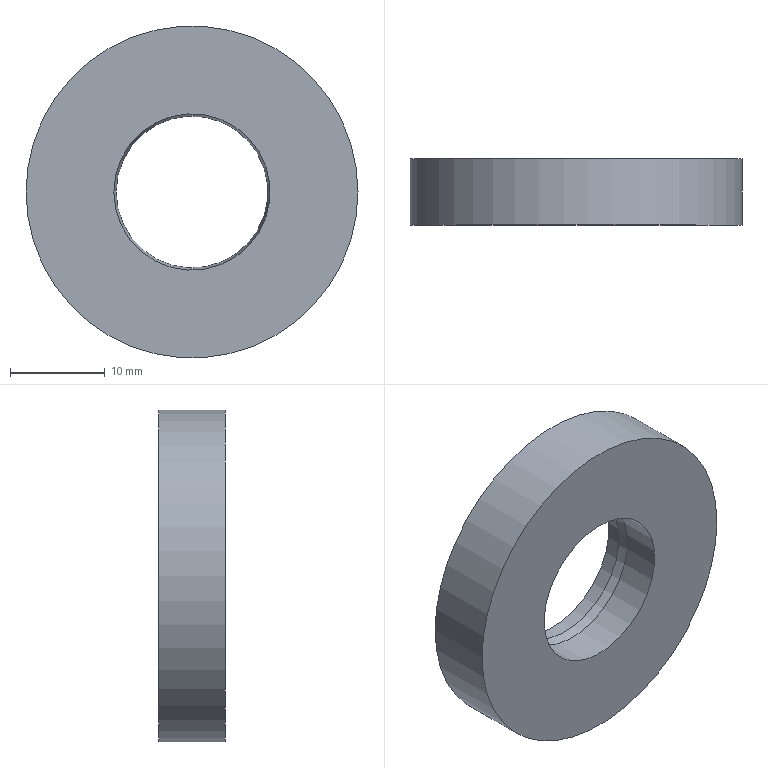Component | NX | OIL_SEAL | 1 solid | 13 faces | box 35 x 7 x 35 mm | volume 2764 mm3 | cylinder 6 | plane 4 | cone 2 | torus 1 | commonest cylinder face diameters 19.32 x2 16.492 x1 35 x1 31.25 x1 16.792 x1
STEP:
#1=CARTESIAN_POINT('',(0.,0.,0.));
#2=DIRECTION('',(0.,0.,1.));
#3=DIRECTION('',(1.,0.,0.));
#4=AXIS2_PLACEMENT_3D('',#1,#2,#3);
#5=CARTESIAN_POINT('',(-8.246,56.,0.));
#6=VERTEX_POINT('',#5);
#7=CARTESIAN_POINT('',(0.,56.,0.));
#8=DIRECTION('',(0.,-1.,0.));
#9=DIRECTION('',(-1.,0.,0.));
#10=AXIS2_PLACEMENT_3D('',#7,#8,#9);
#11=CIRCLE('',#10,8.246);
#12=CARTESIAN_POINT('',(0.,56.,0.));
#13=DIRECTION('',(0.,-1.,0.));
#14=DIRECTION('',(1.,0.,0.));
#15=AXIS2_PLACEMENT_3D('',#12,#13,#14);
#16=CYLINDRICAL_SURFACE('',#15,8.246);
#17=CARTESIAN_POINT('',(3.142,0.));
#18=DIRECTION('',(1.,0.));
#19=VECTOR('',#18,1.);
#20=LINE('',#17,#19);
#21=(GEOMETRIC_REPRESENTATION_CONTEXT(2)PARAMETRIC_REPRESENTATION_CONTEXT()REPRESENTATION_CONTEXT('',''));
#22=DEFINITIONAL_REPRESENTATION('',(#20),#21);
#23=PCURVE('',#16,#22);
#24=CARTESIAN_POINT('',(-8.246,56.,0.));
#25=DIRECTION('',(0.,-1.,0.));
#26=DIRECTION('',(1.,0.,0.));
#27=AXIS2_PLACEMENT_3D('',#24,#25,#26);
#28=PLANE('',#27);
#29=CARTESIAN_POINT('',(8.246,0.));
#30=DIRECTION('',(-1.,0.));
#31=AXIS2_PLACEMENT_2D('',#29,#30);
#32=CIRCLE('',#31,8.246);
#33=(GEOMETRIC_REPRESENTATION_CONTEXT(2)PARAMETRIC_REPRESENTATION_CONTEXT()REPRESENTATION_CONTEXT('',''));
#34=DEFINITIONAL_REPRESENTATION('',(#32),#33);
#35=PCURVE('',#28,#34);
#36=SURFACE_CURVE('',#11,(#23,#35),.PCURVE_S1.);
#37=EDGE_CURVE('',#6,#6,#36,.T.);
#38=ORIENTED_EDGE('',*,*,#37,.F.);
#39=CARTESIAN_POINT('',(-8.246,60.06,0.));
#40=VERTEX_POINT('',#39);
#41=CARTESIAN_POINT('',(-8.246,60.06,0.));
#42=CARTESIAN_POINT('',(-8.246,56.,0.));
#43=B_SPLINE_CURVE_WITH_KNOTS('',1,(#41,#42),.UNSPECIFIED.,.F.,.F.,(2,2),(-4.06,0.),.PIECEWISE_BEZIER_KNOTS.);
#44=CARTESIAN_POINT('',(3.142,0.));
#45=DIRECTION('',(0.,1.));
#46=VECTOR('',#45,1.);
#47=LINE('',#44,#46);
#48=(GEOMETRIC_REPRESENTATION_CONTEXT(2)PARAMETRIC_REPRESENTATION_CONTEXT()REPRESENTATION_CONTEXT('',''));
#49=DEFINITIONAL_REPRESENTATION('',(#47),#48);
#50=PCURVE('',#16,#49);
#51=CARTESIAN_POINT('',(9.425,0.));
#52=DIRECTION('',(0.,1.));
#53=VECTOR('',#52,1.);
#54=LINE('',#51,#53);
#55=(GEOMETRIC_REPRESENTATION_CONTEXT(2)PARAMETRIC_REPRESENTATION_CONTEXT()REPRESENTATION_CONTEXT('',''));
#56=DEFINITIONAL_REPRESENTATION('',(#54),#55);
#57=PCURVE('',#16,#56);
#58=SEAM_CURVE('',#43,(#50,#57),.PCURVE_S1.);
#59=EDGE_CURVE('',#40,#6,#58,.T.);
#60=ORIENTED_EDGE('',*,*,#59,.F.);
#61=CARTESIAN_POINT('',(0.,60.06,0.));
#62=DIRECTION('',(0.,-1.,0.));
#63=DIRECTION('',(-1.,0.,0.));
#64=AXIS2_PLACEMENT_3D('',#61,#62,#63);
#65=CIRCLE('',#64,8.246);
#66=CARTESIAN_POINT('',(3.142,-4.06));
#67=DIRECTION('',(1.,0.));
#68=VECTOR('',#67,1.);
#69=LINE('',#66,#68);
#70=(GEOMETRIC_REPRESENTATION_CONTEXT(2)PARAMETRIC_REPRESENTATION_CONTEXT()REPRESENTATION_CONTEXT('',''));
#71=DEFINITIONAL_REPRESENTATION('',(#69),#70);
#72=PCURVE('',#16,#71);
#73=CARTESIAN_POINT('',(0.,61.106,0.));
#74=DIRECTION('',(0.,-1.,0.));
#75=DIRECTION('',(1.,0.,0.));
#76=AXIS2_PLACEMENT_3D('',#73,#74,#75);
#77=CONICAL_SURFACE('',#76,8.,0.231);
#78=CARTESIAN_POINT('',(3.142,1.046));
#79=DIRECTION('',(1.,0.));
#80=VECTOR('',#79,1.);
#81=LINE('',#78,#80);
#82=(GEOMETRIC_REPRESENTATION_CONTEXT(2)PARAMETRIC_REPRESENTATION_CONTEXT()REPRESENTATION_CONTEXT('',''));
#83=DEFINITIONAL_REPRESENTATION('',(#81),#82);
#84=PCURVE('',#77,#83);
#85=SURFACE_CURVE('',#65,(#72,#84),.PCURVE_S1.);
#86=EDGE_CURVE('',#40,#40,#85,.T.);
#87=ORIENTED_EDGE('',*,*,#86,.T.);
#88=ORIENTED_EDGE('',*,*,#59,.T.);
#89=EDGE_LOOP('',(#38,#60,#87,#88));
#90=FACE_BOUND('',#89,.F.);
#91=ADVANCED_FACE('',(#90),#16,.F.);
#92=CARTESIAN_POINT('',(-17.5,56.,0.));
#93=VERTEX_POINT('',#92);
#94=CARTESIAN_POINT('',(0.,56.,0.));
#95=DIRECTION('',(0.,-1.,0.));
#96=DIRECTION('',(-1.,0.,0.));
#97=AXIS2_PLACEMENT_3D('',#94,#95,#96);
#98=CIRCLE('',#97,17.5);
#99=CARTESIAN_POINT('',(8.246,0.));
#100=DIRECTION('',(-1.,0.));
#101=AXIS2_PLACEMENT_2D('',#99,#100);
#102=CIRCLE('',#101,17.5);
#103=(GEOMETRIC_REPRESENTATION_CONTEXT(2)PARAMETRIC_REPRESENTATION_CONTEXT()REPRESENTATION_CONTEXT('',''));
#104=DEFINITIONAL_REPRESENTATION('',(#102),#103);
#105=PCURVE('',#28,#104);
#106=CARTESIAN_POINT('',(0.,56.,0.));
#107=DIRECTION('',(0.,-1.,0.));
#108=DIRECTION('',(1.,0.,0.));
#109=AXIS2_PLACEMENT_3D('',#106,#107,#108);
#110=CYLINDRICAL_SURFACE('',#109,17.5);
#111=CARTESIAN_POINT('',(3.142,0.));
#112=DIRECTION('',(1.,0.));
#113=VECTOR('',#112,1.);
#114=LINE('',#111,#113);
#115=(GEOMETRIC_REPRESENTATION_CONTEXT(2)PARAMETRIC_REPRESENTATION_CONTEXT()REPRESENTATION_CONTEXT('',''));
#116=DEFINITIONAL_REPRESENTATION('',(#114),#115);
#117=PCURVE('',#110,#116);
#118=SURFACE_CURVE('',#98,(#105,#117),.PCURVE_S1.);
#119=EDGE_CURVE('',#93,#93,#118,.T.);
#120=ORIENTED_EDGE('',*,*,#119,.T.);
#121=EDGE_LOOP('',(#120));
#122=FACE_BOUND('',#121,.T.);
#123=ORIENTED_EDGE('',*,*,#37,.F.);
#124=EDGE_LOOP('',(#123));
#125=FACE_BOUND('',#124,.T.);
#126=ADVANCED_FACE('',(#122,#125),#28,.T.);
#127=CARTESIAN_POINT('',(-17.5,63.,0.));
#128=VERTEX_POINT('',#127);
#129=CARTESIAN_POINT('',(0.,63.,0.));
#130=DIRECTION('',(0.,-1.,0.));
#131=DIRECTION('',(-1.,0.,0.));
#132=AXIS2_PLACEMENT_3D('',#129,#130,#131);
#133=CIRCLE('',#132,17.5);
#134=CARTESIAN_POINT('',(3.142,-7.));
#135=DIRECTION('',(1.,0.));
#136=VECTOR('',#135,1.);
#137=LINE('',#134,#136);
#138=(GEOMETRIC_REPRESENTATION_CONTEXT(2)PARAMETRIC_REPRESENTATION_CONTEXT()REPRESENTATION_CONTEXT('',''));
#139=DEFINITIONAL_REPRESENTATION('',(#137),#138);
#140=PCURVE('',#110,#139);
#141=CARTESIAN_POINT('',(-17.5,63.,0.));
#142=DIRECTION('',(0.,1.,0.));
#143=DIRECTION('',(-1.,0.,0.));
#144=AXIS2_PLACEMENT_3D('',#141,#142,#143);
#145=PLANE('',#144);
#146=CARTESIAN_POINT('',(0.,0.));
#147=CARTESIAN_POINT('',(0.,-30.311));
#148=CARTESIAN_POINT('',(-26.25,-15.155));
#149=CARTESIAN_POINT('',(-52.5,-0.));
#150=CARTESIAN_POINT('',(-26.25,15.155));
#151=CARTESIAN_POINT('',(-0.,30.311));
#152=CARTESIAN_POINT('',(0.,0.));
#153=(BOUNDED_CURVE()B_SPLINE_CURVE(2,(#146,#147,#148,#149,#150,#151,#152),.UNSPECIFIED.,.T.,.F.)B_SPLINE_CURVE_WITH_KNOTS((1,2,2,2,2,1),(-2.094,0.,2.094,4.189,6.283,8.378),.UNSPECIFIED.)CURVE()GEOMETRIC_REPRESENTATION_ITEM()RATIONAL_B_SPLINE_CURVE((1.,0.5,1.,0.5,1.,0.5,1.))REPRESENTATION_ITEM(''));
#154=(GEOMETRIC_REPRESENTATION_CONTEXT(2)PARAMETRIC_REPRESENTATION_CONTEXT()REPRESENTATION_CONTEXT('',''));
#155=DEFINITIONAL_REPRESENTATION('',(#153),#154);
#156=PCURVE('',#145,#155);
#157=SURFACE_CURVE('',#133,(#140,#156),.PCURVE_S1.);
#158=EDGE_CURVE('',#128,#128,#157,.T.);
#159=ORIENTED_EDGE('',*,*,#158,.T.);
#160=CARTESIAN_POINT('',(-17.5,63.,0.));
#161=CARTESIAN_POINT('',(-17.5,56.,0.));
#162=B_SPLINE_CURVE_WITH_KNOTS('',1,(#160,#161),.UNSPECIFIED.,.F.,.F.,(2,2),(-7.,0.),.PIECEWISE_BEZIER_KNOTS.);
#163=CARTESIAN_POINT('',(9.425,0.));
#164=DIRECTION('',(0.,1.));
#165=VECTOR('',#164,1.);
#166=LINE('',#163,#165);
#167=(GEOMETRIC_REPRESENTATION_CONTEXT(2)PARAMETRIC_REPRESENTATION_CONTEXT()REPRESENTATION_CONTEXT('',''));
#168=DEFINITIONAL_REPRESENTATION('',(#166),#167);
#169=PCURVE('',#110,#168);
#170=CARTESIAN_POINT('',(3.142,0.));
#171=DIRECTION('',(0.,1.));
#172=VECTOR('',#171,1.);
#173=LINE('',#170,#172);
#174=(GEOMETRIC_REPRESENTATION_CONTEXT(2)PARAMETRIC_REPRESENTATION_CONTEXT()REPRESENTATION_CONTEXT('',''));
#175=DEFINITIONAL_REPRESENTATION('',(#173),#174);
#176=PCURVE('',#110,#175);
#177=SEAM_CURVE('',#162,(#169,#176),.PCURVE_S1.);
#178=EDGE_CURVE('',#128,#93,#177,.T.);
#179=ORIENTED_EDGE('',*,*,#178,.T.);
#180=ORIENTED_EDGE('',*,*,#119,.F.);
#181=ORIENTED_EDGE('',*,*,#178,.F.);
#182=EDGE_LOOP('',(#159,#179,#180,#181));
#183=FACE_BOUND('',#182,.T.);
#184=ADVANCED_FACE('',(#183),#110,.T.);
#185=CARTESIAN_POINT('',(-15.625,63.,0.));
#186=VERTEX_POINT('',#185);
#187=CARTESIAN_POINT('',(0.,63.,0.));
#188=DIRECTION('',(0.,-1.,0.));
#189=DIRECTION('',(-1.,0.,0.));
#190=AXIS2_PLACEMENT_3D('',#187,#188,#189);
#191=CIRCLE('',#190,15.625);
#192=CARTESIAN_POINT('',(-1.875,0.));
#193=CARTESIAN_POINT('',(-1.875,-27.063));
#194=CARTESIAN_POINT('',(-25.312,-13.532));
#195=CARTESIAN_POINT('',(-48.75,-0.));
#196=CARTESIAN_POINT('',(-25.312,13.532));
#197=CARTESIAN_POINT('',(-1.875,27.063));
#198=CARTESIAN_POINT('',(-1.875,0.));
#199=(BOUNDED_CURVE()B_SPLINE_CURVE(2,(#192,#193,#194,#195,#196,#197,#198),.UNSPECIFIED.,.T.,.F.)B_SPLINE_CURVE_WITH_KNOTS((1,2,2,2,2,1),(-2.094,0.,2.094,4.189,6.283,8.378),.UNSPECIFIED.)CURVE()GEOMETRIC_REPRESENTATION_ITEM()RATIONAL_B_SPLINE_CURVE((1.,0.5,1.,0.5,1.,0.5,1.))REPRESENTATION_ITEM(''));
#200=(GEOMETRIC_REPRESENTATION_CONTEXT(2)PARAMETRIC_REPRESENTATION_CONTEXT()REPRESENTATION_CONTEXT('',''));
#201=DEFINITIONAL_REPRESENTATION('',(#199),#200);
#202=PCURVE('',#145,#201);
#203=CARTESIAN_POINT('',(0.,56.,0.));
#204=DIRECTION('',(0.,-1.,0.));
#205=DIRECTION('',(1.,0.,0.));
#206=AXIS2_PLACEMENT_3D('',#203,#204,#205);
#207=CYLINDRICAL_SURFACE('',#206,15.625);
#208=CARTESIAN_POINT('',(3.142,-7.));
#209=DIRECTION('',(1.,0.));
#210=VECTOR('',#209,1.);
#211=LINE('',#208,#210);
#212=(GEOMETRIC_REPRESENTATION_CONTEXT(2)PARAMETRIC_REPRESENTATION_CONTEXT()REPRESENTATION_CONTEXT('',''));
#213=DEFINITIONAL_REPRESENTATION('',(#211),#212);
#214=PCURVE('',#207,#213);
#215=SURFACE_CURVE('',#191,(#202,#214),.PCURVE_S1.);
#216=EDGE_CURVE('',#186,#186,#215,.T.);
#217=ORIENTED_EDGE('',*,*,#216,.T.);
#218=EDGE_LOOP('',(#217));
#219=FACE_BOUND('',#218,.T.);
#220=ORIENTED_EDGE('',*,*,#158,.F.);
#221=EDGE_LOOP('',(#220));
#222=FACE_BOUND('',#221,.T.);
#223=ADVANCED_FACE('',(#219,#222),#145,.T.);
#224=CARTESIAN_POINT('',(-15.625,57.75,0.));
#225=VERTEX_POINT('',#224);
#226=CARTESIAN_POINT('',(0.,57.75,0.));
#227=DIRECTION('',(0.,-1.,0.));
#228=DIRECTION('',(-1.,0.,0.));
#229=AXIS2_PLACEMENT_3D('',#226,#227,#228);
#230=CIRCLE('',#229,15.625);
#231=CARTESIAN_POINT('',(3.142,-1.75));
#232=DIRECTION('',(1.,0.));
#233=VECTOR('',#232,1.);
#234=LINE('',#231,#233);
#235=(GEOMETRIC_REPRESENTATION_CONTEXT(2)PARAMETRIC_REPRESENTATION_CONTEXT()REPRESENTATION_CONTEXT('',''));
#236=DEFINITIONAL_REPRESENTATION('',(#234),#235);
#237=PCURVE('',#207,#236);
#238=CARTESIAN_POINT('',(-15.625,57.75,0.));
#239=DIRECTION('',(0.,1.,0.));
#240=DIRECTION('',(-1.,0.,0.));
#241=AXIS2_PLACEMENT_3D('',#238,#239,#240);
#242=PLANE('',#241);
#243=CARTESIAN_POINT('',(0.,0.));
#244=CARTESIAN_POINT('',(0.,-27.063));
#245=CARTESIAN_POINT('',(-23.438,-13.532));
#246=CARTESIAN_POINT('',(-46.875,-0.));
#247=CARTESIAN_POINT('',(-23.438,13.532));
#248=CARTESIAN_POINT('',(-0.,27.063));
#249=CARTESIAN_POINT('',(0.,0.));
#250=(BOUNDED_CURVE()B_SPLINE_CURVE(2,(#243,#244,#245,#246,#247,#248,#249),.UNSPECIFIED.,.T.,.F.)B_SPLINE_CURVE_WITH_KNOTS((1,2,2,2,2,1),(-2.094,0.,2.094,4.189,6.283,8.378),.UNSPECIFIED.)CURVE()GEOMETRIC_REPRESENTATION_ITEM()RATIONAL_B_SPLINE_CURVE((1.,0.5,1.,0.5,1.,0.5,1.))REPRESENTATION_ITEM(''));
#251=(GEOMETRIC_REPRESENTATION_CONTEXT(2)PARAMETRIC_REPRESENTATION_CONTEXT()REPRESENTATION_CONTEXT('',''));
#252=DEFINITIONAL_REPRESENTATION('',(#250),#251);
#253=PCURVE('',#242,#252);
#254=SURFACE_CURVE('',#230,(#237,#253),.PCURVE_S1.);
#255=EDGE_CURVE('',#225,#225,#254,.T.);
#256=ORIENTED_EDGE('',*,*,#255,.F.);
#257=CARTESIAN_POINT('',(-15.625,63.,0.));
#258=CARTESIAN_POINT('',(-15.625,57.75,0.));
#259=B_SPLINE_CURVE_WITH_KNOTS('',1,(#257,#258),.UNSPECIFIED.,.F.,.F.,(2,2),(-7.,-1.75),.PIECEWISE_BEZIER_KNOTS.);
#260=CARTESIAN_POINT('',(3.142,0.));
#261=DIRECTION('',(0.,1.));
#262=VECTOR('',#261,1.);
#263=LINE('',#260,#262);
#264=(GEOMETRIC_REPRESENTATION_CONTEXT(2)PARAMETRIC_REPRESENTATION_CONTEXT()REPRESENTATION_CONTEXT('',''));
#265=DEFINITIONAL_REPRESENTATION('',(#263),#264);
#266=PCURVE('',#207,#265);
#267=CARTESIAN_POINT('',(9.425,0.));
#268=DIRECTION('',(0.,1.));
#269=VECTOR('',#268,1.);
#270=LINE('',#267,#269);
#271=(GEOMETRIC_REPRESENTATION_CONTEXT(2)PARAMETRIC_REPRESENTATION_CONTEXT()REPRESENTATION_CONTEXT('',''));
#272=DEFINITIONAL_REPRESENTATION('',(#270),#271);
#273=PCURVE('',#207,#272);
#274=SEAM_CURVE('',#259,(#266,#273),.PCURVE_S1.);
#275=EDGE_CURVE('',#186,#225,#274,.T.);
#276=ORIENTED_EDGE('',*,*,#275,.F.);
#277=ORIENTED_EDGE('',*,*,#216,.T.);
#278=ORIENTED_EDGE('',*,*,#275,.T.);
#279=EDGE_LOOP('',(#256,#276,#277,#278));
#280=FACE_BOUND('',#279,.F.);
#281=ADVANCED_FACE('',(#280),#207,.F.);
#282=CARTESIAN_POINT('',(-9.66,57.75,0.));
#283=VERTEX_POINT('',#282);
#284=CARTESIAN_POINT('',(0.,57.75,0.));
#285=DIRECTION('',(0.,-1.,0.));
#286=DIRECTION('',(-1.,0.,0.));
#287=AXIS2_PLACEMENT_3D('',#284,#285,#286);
#288=CIRCLE('',#287,9.66);
#289=CARTESIAN_POINT('',(-5.965,0.));
#290=CARTESIAN_POINT('',(-5.965,-16.732));
#291=CARTESIAN_POINT('',(-20.455,-8.366));
#292=CARTESIAN_POINT('',(-34.945,-0.));
#293=CARTESIAN_POINT('',(-20.455,8.366));
#294=CARTESIAN_POINT('',(-5.965,16.732));
#295=CARTESIAN_POINT('',(-5.965,0.));
#296=(BOUNDED_CURVE()B_SPLINE_CURVE(2,(#289,#290,#291,#292,#293,#294,#295),.UNSPECIFIED.,.T.,.F.)B_SPLINE_CURVE_WITH_KNOTS((1,2,2,2,2,1),(-2.094,0.,2.094,4.189,6.283,8.378),.UNSPECIFIED.)CURVE()GEOMETRIC_REPRESENTATION_ITEM()RATIONAL_B_SPLINE_CURVE((1.,0.5,1.,0.5,1.,0.5,1.))REPRESENTATION_ITEM(''));
#297=(GEOMETRIC_REPRESENTATION_CONTEXT(2)PARAMETRIC_REPRESENTATION_CONTEXT()REPRESENTATION_CONTEXT('',''));
#298=DEFINITIONAL_REPRESENTATION('',(#296),#297);
#299=PCURVE('',#242,#298);
#300=CARTESIAN_POINT('',(0.,56.,0.));
#301=DIRECTION('',(0.,-1.,0.));
#302=DIRECTION('',(1.,0.,0.));
#303=AXIS2_PLACEMENT_3D('',#300,#301,#302);
#304=CYLINDRICAL_SURFACE('',#303,9.66);
#305=CARTESIAN_POINT('',(3.142,-1.75));
#306=DIRECTION('',(1.,0.));
#307=VECTOR('',#306,1.);
#308=LINE('',#305,#307);
#309=(GEOMETRIC_REPRESENTATION_CONTEXT(2)PARAMETRIC_REPRESENTATION_CONTEXT()REPRESENTATION_CONTEXT('',''));
#310=DEFINITIONAL_REPRESENTATION('',(#308),#309);
#311=PCURVE('',#304,#310);
#312=SURFACE_CURVE('',#288,(#299,#311),.PCURVE_S1.);
#313=EDGE_CURVE('',#283,#283,#312,.T.);
#314=ORIENTED_EDGE('',*,*,#313,.T.);
#315=EDGE_LOOP('',(#314));
#316=FACE_BOUND('',#315,.T.);
#317=ORIENTED_EDGE('',*,*,#255,.F.);
#318=EDGE_LOOP('',(#317));
#319=FACE_BOUND('',#318,.T.);
#320=ADVANCED_FACE('',(#316,#319),#242,.T.);
#321=CARTESIAN_POINT('',(-9.66,61.25,0.));
#322=VERTEX_POINT('',#321);
#323=CARTESIAN_POINT('',(0.,61.25,0.));
#324=DIRECTION('',(0.,-1.,0.));
#325=DIRECTION('',(-1.,0.,0.));
#326=AXIS2_PLACEMENT_3D('',#323,#324,#325);
#327=CIRCLE('',#326,9.66);
#328=CARTESIAN_POINT('',(3.142,-5.25));
#329=DIRECTION('',(1.,0.));
#330=VECTOR('',#329,1.);
#331=LINE('',#328,#330);
#332=(GEOMETRIC_REPRESENTATION_CONTEXT(2)PARAMETRIC_REPRESENTATION_CONTEXT()REPRESENTATION_CONTEXT('',''));
#333=DEFINITIONAL_REPRESENTATION('',(#331),#332);
#334=PCURVE('',#304,#333);
#335=CARTESIAN_POINT('',(0.,61.687,0.));
#336=DIRECTION('',(0.,-1.,0.));
#337=DIRECTION('',(1.,0.,0.));
#338=AXIS2_PLACEMENT_3D('',#335,#336,#337);
#339=TOROIDAL_SURFACE('',#338,9.66,0.4375);
#340=CARTESIAN_POINT('',(3.142,7.854));
#341=DIRECTION('',(1.,0.));
#342=VECTOR('',#341,1.);
#343=LINE('',#340,#342);
#344=(GEOMETRIC_REPRESENTATION_CONTEXT(2)PARAMETRIC_REPRESENTATION_CONTEXT()REPRESENTATION_CONTEXT('',''));
#345=DEFINITIONAL_REPRESENTATION('',(#343),#344);
#346=PCURVE('',#339,#345);
#347=SURFACE_CURVE('',#327,(#334,#346),.PCURVE_S1.);
#348=EDGE_CURVE('',#322,#322,#347,.T.);
#349=ORIENTED_EDGE('',*,*,#348,.T.);
#350=CARTESIAN_POINT('',(-9.66,61.25,0.));
#351=CARTESIAN_POINT('',(-9.66,57.75,0.));
#352=B_SPLINE_CURVE_WITH_KNOTS('',1,(#350,#351),.UNSPECIFIED.,.F.,.F.,(2,2),(-5.25,-1.75),.PIECEWISE_BEZIER_KNOTS.);
#353=CARTESIAN_POINT('',(9.425,0.));
#354=DIRECTION('',(0.,1.));
#355=VECTOR('',#354,1.);
#356=LINE('',#353,#355);
#357=(GEOMETRIC_REPRESENTATION_CONTEXT(2)PARAMETRIC_REPRESENTATION_CONTEXT()REPRESENTATION_CONTEXT('',''));
#358=DEFINITIONAL_REPRESENTATION('',(#356),#357);
#359=PCURVE('',#304,#358);
#360=CARTESIAN_POINT('',(3.142,0.));
#361=DIRECTION('',(0.,1.));
#362=VECTOR('',#361,1.);
#363=LINE('',#360,#362);
#364=(GEOMETRIC_REPRESENTATION_CONTEXT(2)PARAMETRIC_REPRESENTATION_CONTEXT()REPRESENTATION_CONTEXT('',''));
#365=DEFINITIONAL_REPRESENTATION('',(#363),#364);
#366=PCURVE('',#304,#365);
#367=SEAM_CURVE('',#352,(#359,#366),.PCURVE_S1.);
#368=EDGE_CURVE('',#322,#283,#367,.T.);
#369=ORIENTED_EDGE('',*,*,#368,.T.);
#370=ORIENTED_EDGE('',*,*,#313,.F.);
#371=ORIENTED_EDGE('',*,*,#368,.F.);
#372=EDGE_LOOP('',(#349,#369,#370,#371));
#373=FACE_BOUND('',#372,.T.);
#374=ADVANCED_FACE('',(#373),#304,.T.);
#375=CARTESIAN_POINT('',(-9.66,62.125,0.));
#376=VERTEX_POINT('',#375);
#377=CARTESIAN_POINT('',(0.,62.125,0.));
#378=DIRECTION('',(0.,-1.,0.));
#379=DIRECTION('',(-1.,0.,0.));
#380=AXIS2_PLACEMENT_3D('',#377,#378,#379);
#381=CIRCLE('',#380,9.66);
#382=CARTESIAN_POINT('',(3.142,4.712));
#383=DIRECTION('',(1.,0.));
#384=VECTOR('',#383,1.);
#385=LINE('',#382,#384);
#386=(GEOMETRIC_REPRESENTATION_CONTEXT(2)PARAMETRIC_REPRESENTATION_CONTEXT()REPRESENTATION_CONTEXT('',''));
#387=DEFINITIONAL_REPRESENTATION('',(#385),#386);
#388=PCURVE('',#339,#387);
#389=CARTESIAN_POINT('',(0.,56.,0.));
#390=DIRECTION('',(0.,-1.,0.));
#391=DIRECTION('',(1.,0.,0.));
#392=AXIS2_PLACEMENT_3D('',#389,#390,#391);
#393=CYLINDRICAL_SURFACE('',#392,9.66);
#394=CARTESIAN_POINT('',(3.142,-6.125));
#395=DIRECTION('',(1.,0.));
#396=VECTOR('',#395,1.);
#397=LINE('',#394,#396);
#398=(GEOMETRIC_REPRESENTATION_CONTEXT(2)PARAMETRIC_REPRESENTATION_CONTEXT()REPRESENTATION_CONTEXT('',''));
#399=DEFINITIONAL_REPRESENTATION('',(#397),#398);
#400=PCURVE('',#393,#399);
#401=SURFACE_CURVE('',#381,(#388,#400),.PCURVE_S1.);
#402=EDGE_CURVE('',#376,#376,#401,.T.);
#403=ORIENTED_EDGE('',*,*,#402,.T.);
#404=CARTESIAN_POINT('',(-9.66,62.125,0.));
#405=CARTESIAN_POINT('',(-9.856,62.125,0.));
#406=CARTESIAN_POINT('',(-10.053,62.022,0.));
#407=CARTESIAN_POINT('',(-10.185,61.817,0.));
#408=CARTESIAN_POINT('',(-10.185,61.558,0.));
#409=CARTESIAN_POINT('',(-10.053,61.353,0.));
#410=CARTESIAN_POINT('',(-9.856,61.25,0.));
#411=CARTESIAN_POINT('',(-9.66,61.25,0.));
#412=B_SPLINE_CURVE_WITH_KNOTS('',7,(#404,#405,#406,#407,#408,#409,#410,#411),.UNSPECIFIED.,.F.,.F.,(8,8),(4.712,7.854),.PIECEWISE_BEZIER_KNOTS.);
#413=CARTESIAN_POINT('',(9.425,0.));
#414=DIRECTION('',(0.,1.));
#415=VECTOR('',#414,1.);
#416=LINE('',#413,#415);
#417=(GEOMETRIC_REPRESENTATION_CONTEXT(2)PARAMETRIC_REPRESENTATION_CONTEXT()REPRESENTATION_CONTEXT('',''));
#418=DEFINITIONAL_REPRESENTATION('',(#416),#417);
#419=PCURVE('',#339,#418);
#420=CARTESIAN_POINT('',(3.142,0.));
#421=DIRECTION('',(0.,1.));
#422=VECTOR('',#421,1.);
#423=LINE('',#420,#422);
#424=(GEOMETRIC_REPRESENTATION_CONTEXT(2)PARAMETRIC_REPRESENTATION_CONTEXT()REPRESENTATION_CONTEXT('',''));
#425=DEFINITIONAL_REPRESENTATION('',(#423),#424);
#426=PCURVE('',#339,#425);
#427=SEAM_CURVE('',#412,(#419,#426),.PCURVE_S1.);
#428=EDGE_CURVE('',#376,#322,#427,.T.);
#429=ORIENTED_EDGE('',*,*,#428,.T.);
#430=ORIENTED_EDGE('',*,*,#348,.F.);
#431=ORIENTED_EDGE('',*,*,#428,.F.);
#432=EDGE_LOOP('',(#403,#429,#430,#431));
#433=FACE_BOUND('',#432,.T.);
#434=ADVANCED_FACE('',(#433),#339,.T.);
#435=CARTESIAN_POINT('',(-9.66,63.,0.));
#436=VERTEX_POINT('',#435);
#437=CARTESIAN_POINT('',(0.,63.,0.));
#438=DIRECTION('',(0.,-1.,0.));
#439=DIRECTION('',(-1.,0.,0.));
#440=AXIS2_PLACEMENT_3D('',#437,#438,#439);
#441=CIRCLE('',#440,9.66);
#442=CARTESIAN_POINT('',(3.142,-7.));
#443=DIRECTION('',(1.,0.));
#444=VECTOR('',#443,1.);
#445=LINE('',#442,#444);
#446=(GEOMETRIC_REPRESENTATION_CONTEXT(2)PARAMETRIC_REPRESENTATION_CONTEXT()REPRESENTATION_CONTEXT('',''));
#447=DEFINITIONAL_REPRESENTATION('',(#445),#446);
#448=PCURVE('',#393,#447);
#449=CARTESIAN_POINT('',(-9.66,63.,0.));
#450=DIRECTION('',(0.,1.,0.));
#451=DIRECTION('',(-1.,0.,0.));
#452=AXIS2_PLACEMENT_3D('',#449,#450,#451);
#453=PLANE('',#452);
#454=CARTESIAN_POINT('',(0.,0.));
#455=CARTESIAN_POINT('',(0.,-16.732));
#456=CARTESIAN_POINT('',(-14.49,-8.366));
#457=CARTESIAN_POINT('',(-28.98,-0.));
#458=CARTESIAN_POINT('',(-14.49,8.366));
#459=CARTESIAN_POINT('',(-0.,16.732));
#460=CARTESIAN_POINT('',(0.,0.));
#461=(BOUNDED_CURVE()B_SPLINE_CURVE(2,(#454,#455,#456,#457,#458,#459,#460),.UNSPECIFIED.,.T.,.F.)B_SPLINE_CURVE_WITH_KNOTS((1,2,2,2,2,1),(-2.094,0.,2.094,4.189,6.283,8.378),.UNSPECIFIED.)CURVE()GEOMETRIC_REPRESENTATION_ITEM()RATIONAL_B_SPLINE_CURVE((1.,0.5,1.,0.5,1.,0.5,1.))REPRESENTATION_ITEM(''));
#462=(GEOMETRIC_REPRESENTATION_CONTEXT(2)PARAMETRIC_REPRESENTATION_CONTEXT()REPRESENTATION_CONTEXT('',''));
#463=DEFINITIONAL_REPRESENTATION('',(#461),#462);
#464=PCURVE('',#453,#463);
#465=SURFACE_CURVE('',#441,(#448,#464),.PCURVE_S1.);
#466=EDGE_CURVE('',#436,#436,#465,.T.);
#467=ORIENTED_EDGE('',*,*,#466,.T.);
#468=CARTESIAN_POINT('',(-9.66,63.,0.));
#469=CARTESIAN_POINT('',(-9.66,62.125,0.));
#470=B_SPLINE_CURVE_WITH_KNOTS('',1,(#468,#469),.UNSPECIFIED.,.F.,.F.,(2,2),(-7.,-6.125),.PIECEWISE_BEZIER_KNOTS.);
#471=CARTESIAN_POINT('',(9.425,0.));
#472=DIRECTION('',(0.,1.));
#473=VECTOR('',#472,1.);
#474=LINE('',#471,#473);
#475=(GEOMETRIC_REPRESENTATION_CONTEXT(2)PARAMETRIC_REPRESENTATION_CONTEXT()REPRESENTATION_CONTEXT('',''));
#476=DEFINITIONAL_REPRESENTATION('',(#474),#475);
#477=PCURVE('',#393,#476);
#478=CARTESIAN_POINT('',(3.142,0.));
#479=DIRECTION('',(0.,1.));
#480=VECTOR('',#479,1.);
#481=LINE('',#478,#480);
#482=(GEOMETRIC_REPRESENTATION_CONTEXT(2)PARAMETRIC_REPRESENTATION_CONTEXT()REPRESENTATION_CONTEXT('',''));
#483=DEFINITIONAL_REPRESENTATION('',(#481),#482);
#484=PCURVE('',#393,#483);
#485=SEAM_CURVE('',#470,(#477,#484),.PCURVE_S1.);
#486=EDGE_CURVE('',#436,#376,#485,.T.);
#487=ORIENTED_EDGE('',*,*,#486,.T.);
#488=ORIENTED_EDGE('',*,*,#402,.F.);
#489=ORIENTED_EDGE('',*,*,#486,.F.);
#490=EDGE_LOOP('',(#467,#487,#488,#489));
#491=FACE_BOUND('',#490,.T.);
#492=ADVANCED_FACE('',(#491),#393,.T.);
#493=CARTESIAN_POINT('',(-8.396,63.,0.));
#494=VERTEX_POINT('',#493);
#495=CARTESIAN_POINT('',(0.,63.,0.));
#496=DIRECTION('',(0.,-1.,0.));
#497=DIRECTION('',(-1.,0.,0.));
#498=AXIS2_PLACEMENT_3D('',#495,#496,#497);
#499=CIRCLE('',#498,8.396);
#500=CARTESIAN_POINT('',(-1.264,0.));
#501=CARTESIAN_POINT('',(-1.264,-14.542));
#502=CARTESIAN_POINT('',(-13.858,-7.271));
#503=CARTESIAN_POINT('',(-26.452,-0.));
#504=CARTESIAN_POINT('',(-13.858,7.271));
#505=CARTESIAN_POINT('',(-1.264,14.542));
#506=CARTESIAN_POINT('',(-1.264,0.));
#507=(BOUNDED_CURVE()B_SPLINE_CURVE(2,(#500,#501,#502,#503,#504,#505,#506),.UNSPECIFIED.,.T.,.F.)B_SPLINE_CURVE_WITH_KNOTS((1,2,2,2,2,1),(-2.094,0.,2.094,4.189,6.283,8.378),.UNSPECIFIED.)CURVE()GEOMETRIC_REPRESENTATION_ITEM()RATIONAL_B_SPLINE_CURVE((1.,0.5,1.,0.5,1.,0.5,1.))REPRESENTATION_ITEM(''));
#508=(GEOMETRIC_REPRESENTATION_CONTEXT(2)PARAMETRIC_REPRESENTATION_CONTEXT()REPRESENTATION_CONTEXT('',''));
#509=DEFINITIONAL_REPRESENTATION('',(#507),#508);
#510=PCURVE('',#453,#509);
#511=CARTESIAN_POINT('',(0.,56.,0.));
#512=DIRECTION('',(0.,-1.,0.));
#513=DIRECTION('',(1.,0.,0.));
#514=AXIS2_PLACEMENT_3D('',#511,#512,#513);
#515=CYLINDRICAL_SURFACE('',#514,8.396);
#516=CARTESIAN_POINT('',(3.142,-7.));
#517=DIRECTION('',(1.,0.));
#518=VECTOR('',#517,1.);
#519=LINE('',#516,#518);
#520=(GEOMETRIC_REPRESENTATION_CONTEXT(2)PARAMETRIC_REPRESENTATION_CONTEXT()REPRESENTATION_CONTEXT('',''));
#521=DEFINITIONAL_REPRESENTATION('',(#519),#520);
#522=PCURVE('',#515,#521);
#523=SURFACE_CURVE('',#499,(#510,#522),.PCURVE_S1.);
#524=EDGE_CURVE('',#494,#494,#523,.T.);
#525=ORIENTED_EDGE('',*,*,#524,.T.);
#526=EDGE_LOOP('',(#525));
#527=FACE_BOUND('',#526,.T.);
#528=ORIENTED_EDGE('',*,*,#466,.F.);
#529=EDGE_LOOP('',(#528));
#530=FACE_BOUND('',#529,.T.);
#531=ADVANCED_FACE('',(#527,#530),#453,.T.);
#532=CARTESIAN_POINT('',(-8.396,61.25,0.));
#533=VERTEX_POINT('',#532);
#534=CARTESIAN_POINT('',(0.,61.25,0.));
#535=DIRECTION('',(0.,-1.,0.));
#536=DIRECTION('',(-1.,0.,0.));
#537=AXIS2_PLACEMENT_3D('',#534,#535,#536);
#538=CIRCLE('',#537,8.396);
#539=CARTESIAN_POINT('',(3.142,-5.25));
#540=DIRECTION('',(1.,0.));
#541=VECTOR('',#540,1.);
#542=LINE('',#539,#541);
#543=(GEOMETRIC_REPRESENTATION_CONTEXT(2)PARAMETRIC_REPRESENTATION_CONTEXT()REPRESENTATION_CONTEXT('',''));
#544=DEFINITIONAL_REPRESENTATION('',(#542),#543);
#545=PCURVE('',#515,#544);
#546=CARTESIAN_POINT('',(0.,61.25,0.));
#547=DIRECTION('',(0.,1.,0.));
#548=DIRECTION('',(-1.,0.,0.));
#549=AXIS2_PLACEMENT_3D('',#546,#547,#548);
#550=CONICAL_SURFACE('',#549,8.396,1.222);
#551=CARTESIAN_POINT('',(6.283,0.));
#552=DIRECTION('',(-1.,0.));
#553=VECTOR('',#552,1.);
#554=LINE('',#551,#553);
#555=(GEOMETRIC_REPRESENTATION_CONTEXT(2)PARAMETRIC_REPRESENTATION_CONTEXT()REPRESENTATION_CONTEXT('',''));
#556=DEFINITIONAL_REPRESENTATION('',(#554),#555);
#557=PCURVE('',#550,#556);
#558=SURFACE_CURVE('',#538,(#545,#557),.PCURVE_S1.);
#559=EDGE_CURVE('',#533,#533,#558,.T.);
#560=ORIENTED_EDGE('',*,*,#559,.F.);
#561=CARTESIAN_POINT('',(-8.396,63.,0.));
#562=CARTESIAN_POINT('',(-8.396,61.25,0.));
#563=B_SPLINE_CURVE_WITH_KNOTS('',1,(#561,#562),.UNSPECIFIED.,.F.,.F.,(2,2),(-7.,-5.25),.PIECEWISE_BEZIER_KNOTS.);
#564=CARTESIAN_POINT('',(3.142,0.));
#565=DIRECTION('',(0.,1.));
#566=VECTOR('',#565,1.);
#567=LINE('',#564,#566);
#568=(GEOMETRIC_REPRESENTATION_CONTEXT(2)PARAMETRIC_REPRESENTATION_CONTEXT()REPRESENTATION_CONTEXT('',''));
#569=DEFINITIONAL_REPRESENTATION('',(#567),#568);
#570=PCURVE('',#515,#569);
#571=CARTESIAN_POINT('',(9.425,0.));
#572=DIRECTION('',(0.,1.));
#573=VECTOR('',#572,1.);
#574=LINE('',#571,#573);
#575=(GEOMETRIC_REPRESENTATION_CONTEXT(2)PARAMETRIC_REPRESENTATION_CONTEXT()REPRESENTATION_CONTEXT('',''));
#576=DEFINITIONAL_REPRESENTATION('',(#574),#575);
#577=PCURVE('',#515,#576);
#578=SEAM_CURVE('',#563,(#570,#577),.PCURVE_S1.);
#579=EDGE_CURVE('',#494,#533,#578,.T.);
#580=ORIENTED_EDGE('',*,*,#579,.F.);
#581=ORIENTED_EDGE('',*,*,#524,.T.);
#582=ORIENTED_EDGE('',*,*,#579,.T.);
#583=EDGE_LOOP('',(#560,#580,#581,#582));
#584=FACE_BOUND('',#583,.F.);
#585=ADVANCED_FACE('',(#584),#515,.F.);
#586=CARTESIAN_POINT('',(-8.,61.106,0.));
#587=VERTEX_POINT('',#586);
#588=CARTESIAN_POINT('',(0.,61.106,0.));
#589=DIRECTION('',(0.,-1.,0.));
#590=DIRECTION('',(-1.,0.,0.));
#591=AXIS2_PLACEMENT_3D('',#588,#589,#590);
#592=CIRCLE('',#591,8.);
#593=CARTESIAN_POINT('',(6.283,-0.1441));
#594=DIRECTION('',(-1.,0.));
#595=VECTOR('',#594,1.);
#596=LINE('',#593,#595);
#597=(GEOMETRIC_REPRESENTATION_CONTEXT(2)PARAMETRIC_REPRESENTATION_CONTEXT()REPRESENTATION_CONTEXT('',''));
#598=DEFINITIONAL_REPRESENTATION('',(#596),#597);
#599=PCURVE('',#550,#598);
#600=CARTESIAN_POINT('',(3.142,0.));
#601=DIRECTION('',(1.,0.));
#602=VECTOR('',#601,1.);
#603=LINE('',#600,#602);
#604=(GEOMETRIC_REPRESENTATION_CONTEXT(2)PARAMETRIC_REPRESENTATION_CONTEXT()REPRESENTATION_CONTEXT('',''));
#605=DEFINITIONAL_REPRESENTATION('',(#603),#604);
#606=PCURVE('',#77,#605);
#607=SURFACE_CURVE('',#592,(#599,#606),.PCURVE_S1.);
#608=EDGE_CURVE('',#587,#587,#607,.T.);
#609=ORIENTED_EDGE('',*,*,#608,.F.);
#610=CARTESIAN_POINT('',(-8.,61.106,0.));
#611=CARTESIAN_POINT('',(-8.396,61.25,0.));
#612=B_SPLINE_CURVE_WITH_KNOTS('',1,(#610,#611),.UNSPECIFIED.,.F.,.F.,(2,2),(-0.4214,0.),.PIECEWISE_BEZIER_KNOTS.);
#613=CARTESIAN_POINT('',(6.283,0.));
#614=DIRECTION('',(0.,1.));
#615=VECTOR('',#614,1.);
#616=LINE('',#613,#615);
#617=(GEOMETRIC_REPRESENTATION_CONTEXT(2)PARAMETRIC_REPRESENTATION_CONTEXT()REPRESENTATION_CONTEXT('',''));
#618=DEFINITIONAL_REPRESENTATION('',(#616),#617);
#619=PCURVE('',#550,#618);
#620=CARTESIAN_POINT('',(0.,0.));
#621=DIRECTION('',(0.,1.));
#622=VECTOR('',#621,1.);
#623=LINE('',#620,#622);
#624=(GEOMETRIC_REPRESENTATION_CONTEXT(2)PARAMETRIC_REPRESENTATION_CONTEXT()REPRESENTATION_CONTEXT('',''));
#625=DEFINITIONAL_REPRESENTATION('',(#623),#624);
#626=PCURVE('',#550,#625);
#627=SEAM_CURVE('',#612,(#619,#626),.PCURVE_S1.);
#628=EDGE_CURVE('',#587,#533,#627,.T.);
#629=ORIENTED_EDGE('',*,*,#628,.T.);
#630=ORIENTED_EDGE('',*,*,#559,.T.);
#631=ORIENTED_EDGE('',*,*,#628,.F.);
#632=EDGE_LOOP('',(#609,#629,#630,#631));
#633=FACE_BOUND('',#632,.F.);
#634=ADVANCED_FACE('',(#633),#550,.F.);
#635=ORIENTED_EDGE('',*,*,#86,.F.);
#636=CARTESIAN_POINT('',(-8.,61.106,0.));
#637=CARTESIAN_POINT('',(-8.246,60.06,0.));
#638=B_SPLINE_CURVE_WITH_KNOTS('',1,(#636,#637),.UNSPECIFIED.,.F.,.F.,(2,2),(0.,1.074),.PIECEWISE_BEZIER_KNOTS.);
#639=CARTESIAN_POINT('',(3.142,0.));
#640=DIRECTION('',(0.,1.));
#641=VECTOR('',#640,1.);
#642=LINE('',#639,#641);
#643=(GEOMETRIC_REPRESENTATION_CONTEXT(2)PARAMETRIC_REPRESENTATION_CONTEXT()REPRESENTATION_CONTEXT('',''));
#644=DEFINITIONAL_REPRESENTATION('',(#642),#643);
#645=PCURVE('',#77,#644);
#646=CARTESIAN_POINT('',(9.425,0.));
#647=DIRECTION('',(0.,1.));
#648=VECTOR('',#647,1.);
#649=LINE('',#646,#648);
#650=(GEOMETRIC_REPRESENTATION_CONTEXT(2)PARAMETRIC_REPRESENTATION_CONTEXT()REPRESENTATION_CONTEXT('',''));
#651=DEFINITIONAL_REPRESENTATION('',(#649),#650);
#652=PCURVE('',#77,#651);
#653=SEAM_CURVE('',#638,(#645,#652),.PCURVE_S1.);
#654=EDGE_CURVE('',#587,#40,#653,.T.);
#655=ORIENTED_EDGE('',*,*,#654,.F.);
#656=ORIENTED_EDGE('',*,*,#608,.T.);
#657=ORIENTED_EDGE('',*,*,#654,.T.);
#658=EDGE_LOOP('',(#635,#655,#656,#657));
#659=FACE_BOUND('',#658,.F.);
#660=ADVANCED_FACE('',(#659),#77,.F.);
#661=CLOSED_SHELL('',(#91,#126,#184,#223,#281,#320,#374,#434,#492,#531,#585,#634,#660));
#662=MANIFOLD_SOLID_BREP('',#661);
#663=(LENGTH_UNIT()NAMED_UNIT(*)SI_UNIT(.MILLI.,.METRE.));
#664=UNCERTAINTY_MEASURE_WITH_UNIT(LENGTH_MEASURE(0.00001),#663,'','');
#665=(NAMED_UNIT(*)PLANE_ANGLE_UNIT()SI_UNIT($,.RADIAN.));
#666=(NAMED_UNIT(*)SI_UNIT($,.STERADIAN.)SOLID_ANGLE_UNIT());
#667=(GEOMETRIC_REPRESENTATION_CONTEXT(3)GLOBAL_UNCERTAINTY_ASSIGNED_CONTEXT((#664))GLOBAL_UNIT_ASSIGNED_CONTEXT((#663,#665,#666))REPRESENTATION_CONTEXT('',''));
#668=ADVANCED_BREP_SHAPE_REPRESENTATION('',(#4,#662),#667);